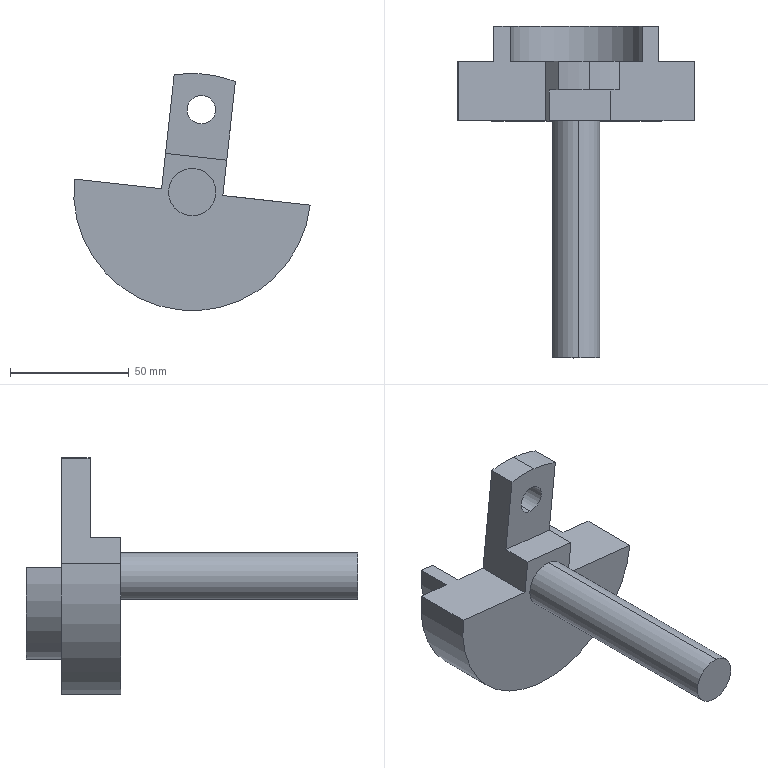Component | SolidWorks | Roller-5 | 1 solid | 20 faces | box 99.7 x 140 x 100 mm | volume 159117 mm3 | plane 11 | cylinder 9 | commonest cylinder face diameters 100 x3 12 x2 20 x2 56 x1 70 x1
build123d program:
from build123d import *

# Parameters (mm, degrees)
SKETCH2_W      = 83.89
SKETCH2_H      = 46.873
EXTRUDE2_DEPTH = 15
SKETCH3_W      = 56.676
SKETCH3_H      = 55.605
EXTRUDE3_DEPTH = 144.614
SKETCH4_R      = 6
EXTRUDE4_DEPTH = 144.614
SKETCH5_W      = 35
SKETCH5_H      = 13
EXTRUDE5_DEPTH = 117.402


with BuildPart() as part:
    # Sketch1 → Revolve1 (revolve)
    with BuildSketch(Plane.XY, mode=Mode.PRIVATE) as revolve1_sk:
        Polygon((0, 69.146), (28, 69.146), (28, 84.146), (35, 84.146), (35, 69.146), (50, 69.146), (50, 44.146), (10, 44.146), (10, -55.854), (0, -55.854), align=None)
    revolve(revolve1_sk.sketch.rotate(Axis((0, 0, 0), (0, 1, 0)), 90), axis=Axis((0, 0, 0), (0, 1, 0)))

    # Sketch2 → Extrude2 (cut)
    with BuildSketch(Plane(origin=(0, 84.146, 0), x_dir=(1, 0, 0), z_dir=(0, 1, 0))):
        with Locations((-6.945, 23.437)):
            Rectangle(SKETCH2_W, SKETCH2_H)
    extrude(amount=-EXTRUDE2_DEPTH, mode=Mode.SUBTRACT)

    # Sketch3 → Extrude3 (cut, through all)
    with BuildSketch(Plane(origin=(0, 69.146, 0), x_dir=(1, 0, 0), z_dir=(0, 1, 0))):
        with Locations((-41.338, 27.803)):
            Rectangle(SKETCH3_W, SKETCH3_H)
        with Locations((41.338, 27.803)):
            Rectangle(SKETCH3_W, SKETCH3_H)
    extrude(amount=-EXTRUDE3_DEPTH, mode=Mode.SUBTRACT)

    # Sketch4 → Extrude4 (cut, through all)
    with BuildSketch(Plane(origin=(0, 69.146, 0), x_dir=(1, 0, 0), z_dir=(0, 1, 0))):
        with Locations(Location((0, 35, 0), (0, 0, 270))):
            Circle(SKETCH4_R)
    extrude(amount=-EXTRUDE4_DEPTH, mode=Mode.SUBTRACT)

    # Sketch5 → Extrude5 (cut, through all)
    with BuildSketch(Plane(origin=(13, 0, 0), x_dir=(0, 0, -1), z_dir=(1, 0, 0))):
        with Locations((32.5, 50.646)):
            Rectangle(SKETCH5_W, SKETCH5_H)
    extrude(amount=-EXTRUDE5_DEPTH, mode=Mode.SUBTRACT)


solid = part.part

# Placed as in the assembly
solid = solid.moved(Location((-214.784, 444.838, 163), (180, -6.299, 180)))
STEP:
#1=COLOUR_RGB('',0.7922,0.8196,0.9333);
#2=FILL_AREA_STYLE_COLOUR('',#1);
#3=FILL_AREA_STYLE('',(#2));
#4=SURFACE_STYLE_FILL_AREA(#3);
#5=SURFACE_SIDE_STYLE('',(#4));
#6=SURFACE_STYLE_USAGE(.BOTH.,#5);
#7=PRESENTATION_STYLE_ASSIGNMENT((#6));
#8=CARTESIAN_POINT('',(-8.331,19.763,7.552));
#9=VERTEX_POINT('',#8);
#10=CARTESIAN_POINT('',(-8.279,19.763,8.022));
#11=VERTEX_POINT('',#10);
#12=CARTESIAN_POINT('',(-8.305,19.763,7.787));
#13=DIRECTION('',(0.,-1.,0.));
#14=DIRECTION('',(-0.1097,0.,-0.994));
#15=AXIS2_PLACEMENT_3D('',#12,#13,#14);
#16=CIRCLE('',#15,0.2362);
#17=EDGE_CURVE('',#9,#11,#16,.T.);
#18=ORIENTED_EDGE('',*,*,#17,.T.);
#19=CARTESIAN_POINT('',(-8.279,20.236,8.022));
#20=VERTEX_POINT('',#19);
#21=CARTESIAN_POINT('',(-8.279,15.314,8.022));
#22=DIRECTION('',(-0.,1.,-0.));
#23=VECTOR('',#22,39.37);
#24=LINE('',#21,#23);
#25=EDGE_CURVE('',#11,#20,#24,.T.);
#26=ORIENTED_EDGE('',*,*,#25,.T.);
#27=CARTESIAN_POINT('',(-8.331,20.236,7.552));
#28=VERTEX_POINT('',#27);
#29=CARTESIAN_POINT('',(-8.305,20.236,7.787));
#30=DIRECTION('',(-0.,1.,-0.));
#31=DIRECTION('',(-0.1097,0.,-0.994));
#32=AXIS2_PLACEMENT_3D('',#29,#30,#31);
#33=CIRCLE('',#32,0.2362);
#34=EDGE_CURVE('',#20,#28,#33,.T.);
#35=ORIENTED_EDGE('',*,*,#34,.T.);
#36=CARTESIAN_POINT('',(-8.331,15.314,7.552));
#37=DIRECTION('',(-0.,1.,-0.));
#38=VECTOR('',#37,39.37);
#39=LINE('',#36,#38);
#40=EDGE_CURVE('',#9,#28,#39,.T.);
#41=ORIENTED_EDGE('',*,*,#40,.F.);
#42=EDGE_LOOP('',(#18,#26,#35,#41));
#43=FACE_OUTER_BOUND('',#42,.T.);
#44=CARTESIAN_POINT('',(-8.305,15.314,7.787));
#45=DIRECTION('',(-0.,1.,-0.));
#46=DIRECTION('',(-0.1097,0.,-0.994));
#47=AXIS2_PLACEMENT_3D('',#44,#45,#46);
#48=CYLINDRICAL_SURFACE('',#47,0.2362);
#49=ADVANCED_FACE('',(#43),#48,.F.);
#50=CARTESIAN_POINT('',(-8.413,19.251,6.809));
#51=VERTEX_POINT('',#50);
#52=CARTESIAN_POINT('',(-8.499,19.251,6.026));
#53=VERTEX_POINT('',#52);
#54=CARTESIAN_POINT('',(-8.456,19.251,6.417));
#55=DIRECTION('',(0.,-1.,0.));
#56=DIRECTION('',(0.1097,0.,0.994));
#57=AXIS2_PLACEMENT_3D('',#54,#55,#56);
#58=CIRCLE('',#57,0.3937);
#59=EDGE_CURVE('',#51,#53,#58,.T.);
#60=ORIENTED_EDGE('',*,*,#59,.T.);
#61=CARTESIAN_POINT('',(-8.499,15.314,6.026));
#62=VERTEX_POINT('',#61);
#63=CARTESIAN_POINT('',(-8.499,17.513,6.026));
#64=DIRECTION('',(0.,-1.,0.));
#65=VECTOR('',#64,39.37);
#66=LINE('',#63,#65);
#67=EDGE_CURVE('',#53,#62,#66,.T.);
#68=ORIENTED_EDGE('',*,*,#67,.T.);
#69=CARTESIAN_POINT('',(-8.413,15.314,6.809));
#70=VERTEX_POINT('',#69);
#71=CARTESIAN_POINT('',(-8.456,15.314,6.417));
#72=DIRECTION('',(0.,-1.,0.));
#73=DIRECTION('',(0.1097,0.,0.994));
#74=AXIS2_PLACEMENT_3D('',#71,#72,#73);
#75=CIRCLE('',#74,0.3937);
#76=EDGE_CURVE('',#70,#62,#75,.T.);
#77=ORIENTED_EDGE('',*,*,#76,.F.);
#78=CARTESIAN_POINT('',(-8.413,17.513,6.809));
#79=DIRECTION('',(0.,-1.,0.));
#80=VECTOR('',#79,39.37);
#81=LINE('',#78,#80);
#82=EDGE_CURVE('',#51,#70,#81,.T.);
#83=ORIENTED_EDGE('',*,*,#82,.F.);
#84=EDGE_LOOP('',(#60,#68,#77,#83));
#85=FACE_OUTER_BOUND('',#84,.T.);
#86=CARTESIAN_POINT('',(-8.456,17.513,6.417));
#87=DIRECTION('',(0.,-1.,0.));
#88=DIRECTION('',(0.1097,0.,0.994));
#89=AXIS2_PLACEMENT_3D('',#86,#87,#88);
#90=CYLINDRICAL_SURFACE('',#89,0.3937);
#91=ADVANCED_FACE('',(#85),#90,.T.);
#92=CARTESIAN_POINT('',(-7.739,20.236,8.25));
#93=VERTEX_POINT('',#92);
#94=CARTESIAN_POINT('',(-8.24,20.236,8.374));
#95=VERTEX_POINT('',#94);
#96=CARTESIAN_POINT('',(-8.456,20.236,6.417));
#97=DIRECTION('',(0.,-1.,0.));
#98=DIRECTION('',(0.1097,0.,0.994));
#99=AXIS2_PLACEMENT_3D('',#96,#97,#98);
#100=CIRCLE('',#99,1.969);
#101=EDGE_CURVE('',#93,#95,#100,.T.);
#102=ORIENTED_EDGE('',*,*,#101,.T.);
#103=CARTESIAN_POINT('',(-8.24,19.763,8.374));
#104=VERTEX_POINT('',#103);
#105=CARTESIAN_POINT('',(-8.24,17.513,8.374));
#106=DIRECTION('',(0.,-1.,0.));
#107=VECTOR('',#106,39.37);
#108=LINE('',#105,#107);
#109=EDGE_CURVE('',#95,#104,#108,.T.);
#110=ORIENTED_EDGE('',*,*,#109,.T.);
#111=CARTESIAN_POINT('',(-7.739,19.763,8.25));
#112=VERTEX_POINT('',#111);
#113=CARTESIAN_POINT('',(-8.456,19.763,6.417));
#114=DIRECTION('',(0.,-1.,0.));
#115=DIRECTION('',(-0.1097,0.,-0.994));
#116=AXIS2_PLACEMENT_3D('',#113,#114,#115);
#117=CIRCLE('',#116,1.969);
#118=EDGE_CURVE('',#112,#104,#117,.T.);
#119=ORIENTED_EDGE('',*,*,#118,.F.);
#120=CARTESIAN_POINT('',(-7.739,17.513,8.25));
#121=DIRECTION('',(0.,-1.,0.));
#122=VECTOR('',#121,39.37);
#123=LINE('',#120,#122);
#124=EDGE_CURVE('',#93,#112,#123,.T.);
#125=ORIENTED_EDGE('',*,*,#124,.F.);
#126=EDGE_LOOP('',(#102,#110,#119,#125));
#127=FACE_OUTER_BOUND('',#126,.T.);
#128=CARTESIAN_POINT('',(-8.456,17.513,6.417));
#129=DIRECTION('',(0.,-1.,0.));
#130=DIRECTION('',(0.1097,0.,0.994));
#131=AXIS2_PLACEMENT_3D('',#128,#129,#130);
#132=CYLINDRICAL_SURFACE('',#131,1.969);
#133=ADVANCED_FACE('',(#127),#132,.T.);
#134=CARTESIAN_POINT('',(-9.826,20.236,6.569));
#135=VERTEX_POINT('',#134);
#136=CARTESIAN_POINT('',(-10.413,20.236,6.633));
#137=VERTEX_POINT('',#136);
#138=CARTESIAN_POINT('',(-11.183,20.236,6.718));
#139=DIRECTION('',(-0.994,-0.,0.1097));
#140=VECTOR('',#139,39.37);
#141=LINE('',#138,#140);
#142=EDGE_CURVE('',#135,#137,#141,.T.);
#143=ORIENTED_EDGE('',*,*,#142,.F.);
#144=CARTESIAN_POINT('',(-7.086,20.236,6.266));
#145=VERTEX_POINT('',#144);
#146=CARTESIAN_POINT('',(-8.456,20.236,6.417));
#147=DIRECTION('',(0.,-1.,0.));
#148=DIRECTION('',(0.1097,0.,0.994));
#149=AXIS2_PLACEMENT_3D('',#146,#147,#148);
#150=CIRCLE('',#149,1.378);
#151=EDGE_CURVE('',#135,#145,#150,.T.);
#152=ORIENTED_EDGE('',*,*,#151,.T.);
#153=CARTESIAN_POINT('',(-6.499,20.236,6.201));
#154=VERTEX_POINT('',#153);
#155=CARTESIAN_POINT('',(-5.729,20.236,6.116));
#156=DIRECTION('',(-0.994,-0.,0.1097));
#157=VECTOR('',#156,39.37);
#158=LINE('',#155,#157);
#159=EDGE_CURVE('',#154,#145,#158,.T.);
#160=ORIENTED_EDGE('',*,*,#159,.F.);
#161=CARTESIAN_POINT('',(-8.456,20.236,6.417));
#162=DIRECTION('',(0.,-1.,0.));
#163=DIRECTION('',(0.1097,0.,0.994));
#164=AXIS2_PLACEMENT_3D('',#161,#162,#163);
#165=CIRCLE('',#164,1.969);
#166=EDGE_CURVE('',#137,#154,#165,.T.);
#167=ORIENTED_EDGE('',*,*,#166,.F.);
#168=EDGE_LOOP('',(#143,#152,#160,#167));
#169=FACE_OUTER_BOUND('',#168,.T.);
#170=CARTESIAN_POINT('',(-9.826,20.236,6.569));
#171=DIRECTION('',(-0.,1.,-0.));
#172=DIRECTION('',(-0.1097,-0.,-0.994));
#173=AXIS2_PLACEMENT_3D('',#170,#171,#172);
#174=PLANE('',#173);
#175=ADVANCED_FACE('',(#169),#174,.T.);
#176=CARTESIAN_POINT('',(-10.413,19.251,6.633));
#177=VERTEX_POINT('',#176);
#178=CARTESIAN_POINT('',(-10.413,17.513,6.633));
#179=DIRECTION('',(0.,-1.,0.));
#180=VECTOR('',#179,39.37);
#181=LINE('',#178,#180);
#182=EDGE_CURVE('',#137,#177,#181,.T.);
#183=ORIENTED_EDGE('',*,*,#182,.F.);
#184=ORIENTED_EDGE('',*,*,#166,.T.);
#185=CARTESIAN_POINT('',(-6.499,19.251,6.201));
#186=VERTEX_POINT('',#185);
#187=CARTESIAN_POINT('',(-6.499,17.513,6.201));
#188=DIRECTION('',(-0.,1.,-0.));
#189=VECTOR('',#188,39.37);
#190=LINE('',#187,#189);
#191=EDGE_CURVE('',#186,#154,#190,.T.);
#192=ORIENTED_EDGE('',*,*,#191,.F.);
#193=CARTESIAN_POINT('',(-8.456,19.251,6.417));
#194=DIRECTION('',(0.,-1.,0.));
#195=DIRECTION('',(0.1097,0.,0.994));
#196=AXIS2_PLACEMENT_3D('',#193,#194,#195);
#197=CIRCLE('',#196,1.969);
#198=EDGE_CURVE('',#177,#186,#197,.T.);
#199=ORIENTED_EDGE('',*,*,#198,.F.);
#200=EDGE_LOOP('',(#183,#184,#192,#199));
#201=FACE_OUTER_BOUND('',#200,.T.);
#202=CARTESIAN_POINT('',(-8.456,17.513,6.417));
#203=DIRECTION('',(0.,-1.,0.));
#204=DIRECTION('',(0.1097,0.,0.994));
#205=AXIS2_PLACEMENT_3D('',#202,#203,#204);
#206=CYLINDRICAL_SURFACE('',#205,1.969);
#207=ADVANCED_FACE('',(#201),#206,.T.);
#208=CARTESIAN_POINT('',(-7.36,20.826,6.296));
#209=VERTEX_POINT('',#208);
#210=CARTESIAN_POINT('',(-7.36,20.236,6.296));
#211=VERTEX_POINT('',#210);
#212=CARTESIAN_POINT('',(-7.36,17.513,6.296));
#213=DIRECTION('',(0.,-1.,0.));
#214=VECTOR('',#213,39.37);
#215=LINE('',#212,#214);
#216=EDGE_CURVE('',#209,#211,#215,.T.);
#217=ORIENTED_EDGE('',*,*,#216,.F.);
#218=CARTESIAN_POINT('',(-9.552,20.826,6.538));
#219=VERTEX_POINT('',#218);
#220=CARTESIAN_POINT('',(-8.456,20.826,6.417));
#221=DIRECTION('',(0.,-1.,0.));
#222=DIRECTION('',(0.1097,0.,0.994));
#223=AXIS2_PLACEMENT_3D('',#220,#221,#222);
#224=CIRCLE('',#223,1.102);
#225=EDGE_CURVE('',#219,#209,#224,.T.);
#226=ORIENTED_EDGE('',*,*,#225,.F.);
#227=CARTESIAN_POINT('',(-9.552,20.236,6.538));
#228=VERTEX_POINT('',#227);
#229=CARTESIAN_POINT('',(-9.552,17.513,6.538));
#230=DIRECTION('',(-0.,1.,-0.));
#231=VECTOR('',#230,39.37);
#232=LINE('',#229,#231);
#233=EDGE_CURVE('',#228,#219,#232,.T.);
#234=ORIENTED_EDGE('',*,*,#233,.F.);
#235=CARTESIAN_POINT('',(-8.456,20.236,6.417));
#236=DIRECTION('',(0.,-1.,0.));
#237=DIRECTION('',(0.1097,0.,0.994));
#238=AXIS2_PLACEMENT_3D('',#235,#236,#237);
#239=CIRCLE('',#238,1.102);
#240=EDGE_CURVE('',#228,#211,#239,.T.);
#241=ORIENTED_EDGE('',*,*,#240,.T.);
#242=EDGE_LOOP('',(#217,#226,#234,#241));
#243=FACE_OUTER_BOUND('',#242,.T.);
#244=CARTESIAN_POINT('',(-8.456,17.513,6.417));
#245=DIRECTION('',(0.,-1.,0.));
#246=DIRECTION('',(0.1097,0.,0.994));
#247=AXIS2_PLACEMENT_3D('',#244,#245,#246);
#248=CYLINDRICAL_SURFACE('',#247,1.102);
#249=ADVANCED_FACE('',(#243),#248,.F.);
#250=CARTESIAN_POINT('',(-7.086,20.826,6.266));
#251=VERTEX_POINT('',#250);
#252=CARTESIAN_POINT('',(-6.543,20.826,6.206));
#253=DIRECTION('',(-0.994,-0.,0.1097));
#254=VECTOR('',#253,39.37);
#255=LINE('',#252,#254);
#256=EDGE_CURVE('',#251,#209,#255,.T.);
#257=ORIENTED_EDGE('',*,*,#256,.F.);
#258=CARTESIAN_POINT('',(-9.826,20.826,6.569));
#259=VERTEX_POINT('',#258);
#260=CARTESIAN_POINT('',(-8.456,20.826,6.417));
#261=DIRECTION('',(0.,-1.,0.));
#262=DIRECTION('',(0.1097,0.,0.994));
#263=AXIS2_PLACEMENT_3D('',#260,#261,#262);
#264=CIRCLE('',#263,1.378);
#265=EDGE_CURVE('',#259,#251,#264,.T.);
#266=ORIENTED_EDGE('',*,*,#265,.F.);
#267=CARTESIAN_POINT('',(-6.543,20.826,6.206));
#268=DIRECTION('',(-0.994,-0.,0.1097));
#269=VECTOR('',#268,39.37);
#270=LINE('',#267,#269);
#271=EDGE_CURVE('',#219,#259,#270,.T.);
#272=ORIENTED_EDGE('',*,*,#271,.F.);
#273=ORIENTED_EDGE('',*,*,#225,.T.);
#274=EDGE_LOOP('',(#257,#266,#272,#273));
#275=FACE_OUTER_BOUND('',#274,.T.);
#276=CARTESIAN_POINT('',(-9.552,20.826,6.538));
#277=DIRECTION('',(-0.,1.,-0.));
#278=DIRECTION('',(-0.1097,-0.,-0.994));
#279=AXIS2_PLACEMENT_3D('',#276,#277,#278);
#280=PLANE('',#279);
#281=ADVANCED_FACE('',(#275),#280,.T.);
#282=CARTESIAN_POINT('',(-7.086,17.513,6.266));
#283=DIRECTION('',(-0.,1.,-0.));
#284=VECTOR('',#283,39.37);
#285=LINE('',#282,#284);
#286=EDGE_CURVE('',#145,#251,#285,.T.);
#287=ORIENTED_EDGE('',*,*,#286,.F.);
#288=ORIENTED_EDGE('',*,*,#151,.F.);
#289=CARTESIAN_POINT('',(-9.826,16.452,6.569));
#290=DIRECTION('',(-0.,1.,-0.));
#291=VECTOR('',#290,39.37);
#292=LINE('',#289,#291);
#293=EDGE_CURVE('',#135,#259,#292,.T.);
#294=ORIENTED_EDGE('',*,*,#293,.T.);
#295=ORIENTED_EDGE('',*,*,#265,.T.);
#296=EDGE_LOOP('',(#287,#288,#294,#295));
#297=FACE_OUTER_BOUND('',#296,.T.);
#298=CARTESIAN_POINT('',(-8.456,17.513,6.417));
#299=DIRECTION('',(0.,-1.,0.));
#300=DIRECTION('',(0.1097,0.,0.994));
#301=AXIS2_PLACEMENT_3D('',#298,#299,#300);
#302=CYLINDRICAL_SURFACE('',#301,1.378);
#303=ADVANCED_FACE('',(#297),#302,.T.);
#304=CARTESIAN_POINT('',(-8.305,20.236,7.787));
#305=DIRECTION('',(-0.,1.,-0.));
#306=DIRECTION('',(-0.1097,0.,-0.994));
#307=AXIS2_PLACEMENT_3D('',#304,#305,#306);
#308=CIRCLE('',#307,0.2362);
#309=EDGE_CURVE('',#28,#20,#308,.T.);
#310=ORIENTED_EDGE('',*,*,#309,.F.);
#311=ORIENTED_EDGE('',*,*,#34,.F.);
#312=EDGE_LOOP('',(#310,#311));
#313=FACE_BOUND('',#312,.T.);
#314=CARTESIAN_POINT('',(-8.965,20.236,6.473));
#315=VERTEX_POINT('',#314);
#316=CARTESIAN_POINT('',(-11.183,20.236,6.718));
#317=DIRECTION('',(-0.994,-0.,0.1097));
#318=VECTOR('',#317,39.37);
#319=LINE('',#316,#318);
#320=EDGE_CURVE('',#315,#228,#319,.T.);
#321=ORIENTED_EDGE('',*,*,#320,.F.);
#322=CARTESIAN_POINT('',(-8.756,20.236,8.363));
#323=VERTEX_POINT('',#322);
#324=CARTESIAN_POINT('',(-8.725,20.236,8.649));
#325=DIRECTION('',(-0.1097,-0.,-0.994));
#326=VECTOR('',#325,39.37);
#327=LINE('',#324,#326);
#328=EDGE_CURVE('',#323,#315,#327,.T.);
#329=ORIENTED_EDGE('',*,*,#328,.F.);
#330=CARTESIAN_POINT('',(-8.456,20.236,6.417));
#331=DIRECTION('',(0.,-1.,0.));
#332=DIRECTION('',(0.1097,0.,0.994));
#333=AXIS2_PLACEMENT_3D('',#330,#331,#332);
#334=CIRCLE('',#333,1.969);
#335=EDGE_CURVE('',#95,#323,#334,.T.);
#336=ORIENTED_EDGE('',*,*,#335,.F.);
#337=ORIENTED_EDGE('',*,*,#101,.F.);
#338=CARTESIAN_POINT('',(-7.947,20.236,6.361));
#339=VERTEX_POINT('',#338);
#340=CARTESIAN_POINT('',(-7.707,20.236,8.537));
#341=DIRECTION('',(0.1097,0.,0.994));
#342=VECTOR('',#341,39.37);
#343=LINE('',#340,#342);
#344=EDGE_CURVE('',#339,#93,#343,.T.);
#345=ORIENTED_EDGE('',*,*,#344,.F.);
#346=CARTESIAN_POINT('',(-5.729,20.236,6.116));
#347=DIRECTION('',(-0.994,-0.,0.1097));
#348=VECTOR('',#347,39.37);
#349=LINE('',#346,#348);
#350=EDGE_CURVE('',#211,#339,#349,.T.);
#351=ORIENTED_EDGE('',*,*,#350,.F.);
#352=ORIENTED_EDGE('',*,*,#240,.F.);
#353=EDGE_LOOP('',(#321,#329,#336,#337,#345,#351,#352));
#354=FACE_OUTER_BOUND('',#353,.T.);
#355=CARTESIAN_POINT('',(-9.826,20.236,6.569));
#356=DIRECTION('',(-0.,1.,-0.));
#357=DIRECTION('',(-0.1097,-0.,-0.994));
#358=AXIS2_PLACEMENT_3D('',#355,#356,#357);
#359=PLANE('',#358);
#360=ADVANCED_FACE('',(#313,#354),#359,.T.);
#361=ORIENTED_EDGE('',*,*,#109,.F.);
#362=ORIENTED_EDGE('',*,*,#335,.T.);
#363=CARTESIAN_POINT('',(-8.756,19.763,8.363));
#364=VERTEX_POINT('',#363);
#365=CARTESIAN_POINT('',(-8.756,17.513,8.363));
#366=DIRECTION('',(-0.,1.,-0.));
#367=VECTOR('',#366,39.37);
#368=LINE('',#365,#367);
#369=EDGE_CURVE('',#364,#323,#368,.T.);
#370=ORIENTED_EDGE('',*,*,#369,.F.);
#371=CARTESIAN_POINT('',(-8.456,19.763,6.417));
#372=DIRECTION('',(0.,-1.,0.));
#373=DIRECTION('',(-0.1097,0.,-0.994));
#374=AXIS2_PLACEMENT_3D('',#371,#372,#373);
#375=CIRCLE('',#374,1.969);
#376=EDGE_CURVE('',#104,#364,#375,.T.);
#377=ORIENTED_EDGE('',*,*,#376,.F.);
#378=EDGE_LOOP('',(#361,#362,#370,#377));
#379=FACE_OUTER_BOUND('',#378,.T.);
#380=CARTESIAN_POINT('',(-8.456,17.513,6.417));
#381=DIRECTION('',(0.,-1.,0.));
#382=DIRECTION('',(0.1097,0.,0.994));
#383=AXIS2_PLACEMENT_3D('',#380,#381,#382);
#384=CYLINDRICAL_SURFACE('',#383,1.969);
#385=ADVANCED_FACE('',(#379),#384,.T.);
#386=CARTESIAN_POINT('',(-7.883,19.251,6.948));
#387=VERTEX_POINT('',#386);
#388=CARTESIAN_POINT('',(-8.9,19.251,7.06));
#389=VERTEX_POINT('',#388);
#390=CARTESIAN_POINT('',(-6.435,19.251,6.788));
#391=DIRECTION('',(-0.994,-0.,0.1097));
#392=VECTOR('',#391,39.37);
#393=LINE('',#390,#392);
#394=EDGE_CURVE('',#387,#389,#393,.T.);
#395=ORIENTED_EDGE('',*,*,#394,.T.);
#396=CARTESIAN_POINT('',(-8.965,19.251,6.473));
#397=VERTEX_POINT('',#396);
#398=CARTESIAN_POINT('',(-8.965,19.251,6.473));
#399=DIRECTION('',(0.1097,0.,0.994));
#400=VECTOR('',#399,39.37);
#401=LINE('',#398,#400);
#402=EDGE_CURVE('',#397,#389,#401,.T.);
#403=ORIENTED_EDGE('',*,*,#402,.F.);
#404=CARTESIAN_POINT('',(-10.413,19.251,6.633));
#405=DIRECTION('',(0.994,0.,-0.1097));
#406=VECTOR('',#405,39.37);
#407=LINE('',#404,#406);
#408=EDGE_CURVE('',#177,#397,#407,.T.);
#409=ORIENTED_EDGE('',*,*,#408,.F.);
#410=ORIENTED_EDGE('',*,*,#198,.T.);
#411=CARTESIAN_POINT('',(-7.947,19.251,6.361));
#412=VERTEX_POINT('',#411);
#413=CARTESIAN_POINT('',(-10.413,19.251,6.633));
#414=DIRECTION('',(0.994,0.,-0.1097));
#415=VECTOR('',#414,39.37);
#416=LINE('',#413,#415);
#417=EDGE_CURVE('',#412,#186,#416,.T.);
#418=ORIENTED_EDGE('',*,*,#417,.F.);
#419=CARTESIAN_POINT('',(-7.947,19.251,6.361));
#420=DIRECTION('',(-0.1097,-0.,-0.994));
#421=VECTOR('',#420,39.37);
#422=LINE('',#419,#421);
#423=EDGE_CURVE('',#387,#412,#422,.T.);
#424=ORIENTED_EDGE('',*,*,#423,.F.);
#425=EDGE_LOOP('',(#395,#403,#409,#410,#418,#424));
#426=FACE_OUTER_BOUND('',#425,.T.);
#427=ORIENTED_EDGE('',*,*,#59,.F.);
#428=CARTESIAN_POINT('',(-8.456,19.251,6.417));
#429=DIRECTION('',(0.,-1.,0.));
#430=DIRECTION('',(0.1097,0.,0.994));
#431=AXIS2_PLACEMENT_3D('',#428,#429,#430);
#432=CIRCLE('',#431,0.3937);
#433=EDGE_CURVE('',#53,#51,#432,.T.);
#434=ORIENTED_EDGE('',*,*,#433,.F.);
#435=EDGE_LOOP('',(#427,#434));
#436=FACE_BOUND('',#435,.T.);
#437=CARTESIAN_POINT('',(-10.413,19.251,6.633));
#438=DIRECTION('',(0.,-1.,0.));
#439=DIRECTION('',(0.1097,0.,0.994));
#440=AXIS2_PLACEMENT_3D('',#437,#438,#439);
#441=PLANE('',#440);
#442=ADVANCED_FACE('',(#426,#436),#441,.T.);
#443=ORIENTED_EDGE('',*,*,#67,.F.);
#444=ORIENTED_EDGE('',*,*,#433,.T.);
#445=ORIENTED_EDGE('',*,*,#82,.T.);
#446=CARTESIAN_POINT('',(-8.456,15.314,6.417));
#447=DIRECTION('',(0.,-1.,0.));
#448=DIRECTION('',(0.1097,0.,0.994));
#449=AXIS2_PLACEMENT_3D('',#446,#447,#448);
#450=CIRCLE('',#449,0.3937);
#451=EDGE_CURVE('',#62,#70,#450,.T.);
#452=ORIENTED_EDGE('',*,*,#451,.F.);
#453=EDGE_LOOP('',(#443,#444,#445,#452));
#454=FACE_OUTER_BOUND('',#453,.T.);
#455=CARTESIAN_POINT('',(-8.456,17.513,6.417));
#456=DIRECTION('',(0.,-1.,0.));
#457=DIRECTION('',(0.1097,0.,0.994));
#458=AXIS2_PLACEMENT_3D('',#455,#456,#457);
#459=CYLINDRICAL_SURFACE('',#458,0.3937);
#460=ADVANCED_FACE('',(#454),#459,.T.);
#461=ORIENTED_EDGE('',*,*,#76,.T.);
#462=ORIENTED_EDGE('',*,*,#451,.T.);
#463=EDGE_LOOP('',(#461,#462));
#464=FACE_OUTER_BOUND('',#463,.T.);
#465=CARTESIAN_POINT('',(-8.847,15.314,6.461));
#466=DIRECTION('',(0.,-1.,0.));
#467=DIRECTION('',(0.1097,0.,0.994));
#468=AXIS2_PLACEMENT_3D('',#465,#466,#467);
#469=PLANE('',#468);
#470=ADVANCED_FACE('',(#464),#469,.T.);
#471=ORIENTED_EDGE('',*,*,#216,.T.);
#472=ORIENTED_EDGE('',*,*,#350,.T.);
#473=CARTESIAN_POINT('',(-7.947,15.314,6.361));
#474=DIRECTION('',(-0.,1.,-0.));
#475=VECTOR('',#474,39.37);
#476=LINE('',#473,#475);
#477=EDGE_CURVE('',#412,#339,#476,.T.);
#478=ORIENTED_EDGE('',*,*,#477,.F.);
#479=ORIENTED_EDGE('',*,*,#417,.T.);
#480=ORIENTED_EDGE('',*,*,#191,.T.);
#481=ORIENTED_EDGE('',*,*,#159,.T.);
#482=ORIENTED_EDGE('',*,*,#286,.T.);
#483=ORIENTED_EDGE('',*,*,#256,.T.);
#484=EDGE_LOOP('',(#471,#472,#478,#479,#480,#481,#482,#483));
#485=FACE_OUTER_BOUND('',#484,.T.);
#486=CARTESIAN_POINT('',(-6.543,16.452,6.206));
#487=DIRECTION('',(-0.1097,-0.,-0.994));
#488=DIRECTION('',(-0.994,-0.,0.1097));
#489=AXIS2_PLACEMENT_3D('',#486,#487,#488);
#490=PLANE('',#489);
#491=ADVANCED_FACE('',(#485),#490,.F.);
#492=ORIENTED_EDGE('',*,*,#233,.T.);
#493=ORIENTED_EDGE('',*,*,#271,.T.);
#494=ORIENTED_EDGE('',*,*,#293,.F.);
#495=ORIENTED_EDGE('',*,*,#142,.T.);
#496=ORIENTED_EDGE('',*,*,#182,.T.);
#497=ORIENTED_EDGE('',*,*,#408,.T.);
#498=CARTESIAN_POINT('',(-8.965,15.314,6.473));
#499=DIRECTION('',(-0.,1.,-0.));
#500=VECTOR('',#499,39.37);
#501=LINE('',#498,#500);
#502=EDGE_CURVE('',#397,#315,#501,.T.);
#503=ORIENTED_EDGE('',*,*,#502,.T.);
#504=ORIENTED_EDGE('',*,*,#320,.T.);
#505=EDGE_LOOP('',(#492,#493,#494,#495,#496,#497,#503,#504));
#506=FACE_OUTER_BOUND('',#505,.T.);
#507=CARTESIAN_POINT('',(-6.543,16.452,6.206));
#508=DIRECTION('',(-0.1097,-0.,-0.994));
#509=DIRECTION('',(-0.994,-0.,0.1097));
#510=AXIS2_PLACEMENT_3D('',#507,#508,#509);
#511=PLANE('',#510);
#512=ADVANCED_FACE('',(#506),#511,.F.);
#513=CARTESIAN_POINT('',(-7.883,19.763,6.948));
#514=VERTEX_POINT('',#513);
#515=CARTESIAN_POINT('',(-7.707,19.763,8.537));
#516=DIRECTION('',(-0.1097,-0.,-0.994));
#517=VECTOR('',#516,39.37);
#518=LINE('',#515,#517);
#519=EDGE_CURVE('',#112,#514,#518,.T.);
#520=ORIENTED_EDGE('',*,*,#519,.T.);
#521=CARTESIAN_POINT('',(-7.883,15.314,6.948));
#522=DIRECTION('',(0.,-1.,0.));
#523=VECTOR('',#522,39.37);
#524=LINE('',#521,#523);
#525=EDGE_CURVE('',#514,#387,#524,.T.);
#526=ORIENTED_EDGE('',*,*,#525,.T.);
#527=ORIENTED_EDGE('',*,*,#423,.T.);
#528=ORIENTED_EDGE('',*,*,#477,.T.);
#529=ORIENTED_EDGE('',*,*,#344,.T.);
#530=ORIENTED_EDGE('',*,*,#124,.T.);
#531=EDGE_LOOP('',(#520,#526,#527,#528,#529,#530));
#532=FACE_OUTER_BOUND('',#531,.T.);
#533=CARTESIAN_POINT('',(-7.707,15.314,8.537));
#534=DIRECTION('',(-0.994,-0.,0.1097));
#535=DIRECTION('',(0.1097,0.,0.994));
#536=AXIS2_PLACEMENT_3D('',#533,#534,#535);
#537=PLANE('',#536);
#538=ADVANCED_FACE('',(#532),#537,.F.);
#539=ORIENTED_EDGE('',*,*,#402,.T.);
#540=CARTESIAN_POINT('',(-8.9,19.763,7.06));
#541=VERTEX_POINT('',#540);
#542=CARTESIAN_POINT('',(-8.9,19.251,7.06));
#543=DIRECTION('',(0.,-1.,0.));
#544=VECTOR('',#543,39.37);
#545=LINE('',#542,#544);
#546=EDGE_CURVE('',#541,#389,#545,.T.);
#547=ORIENTED_EDGE('',*,*,#546,.F.);
#548=CARTESIAN_POINT('',(-8.749,19.763,8.43));
#549=DIRECTION('',(-0.1097,-0.,-0.994));
#550=VECTOR('',#549,39.37);
#551=LINE('',#548,#550);
#552=EDGE_CURVE('',#364,#541,#551,.T.);
#553=ORIENTED_EDGE('',*,*,#552,.F.);
#554=ORIENTED_EDGE('',*,*,#369,.T.);
#555=ORIENTED_EDGE('',*,*,#328,.T.);
#556=ORIENTED_EDGE('',*,*,#502,.F.);
#557=EDGE_LOOP('',(#539,#547,#553,#554,#555,#556));
#558=FACE_OUTER_BOUND('',#557,.T.);
#559=CARTESIAN_POINT('',(-8.725,15.314,8.649));
#560=DIRECTION('',(0.994,0.,-0.1097));
#561=DIRECTION('',(-0.1097,-0.,-0.994));
#562=AXIS2_PLACEMENT_3D('',#559,#560,#561);
#563=PLANE('',#562);
#564=ADVANCED_FACE('',(#558),#563,.F.);
#565=ORIENTED_EDGE('',*,*,#25,.F.);
#566=CARTESIAN_POINT('',(-8.305,19.763,7.787));
#567=DIRECTION('',(0.,-1.,0.));
#568=DIRECTION('',(-0.1097,0.,-0.994));
#569=AXIS2_PLACEMENT_3D('',#566,#567,#568);
#570=CIRCLE('',#569,0.2362);
#571=EDGE_CURVE('',#11,#9,#570,.T.);
#572=ORIENTED_EDGE('',*,*,#571,.T.);
#573=ORIENTED_EDGE('',*,*,#40,.T.);
#574=ORIENTED_EDGE('',*,*,#309,.T.);
#575=EDGE_LOOP('',(#565,#572,#573,#574));
#576=FACE_OUTER_BOUND('',#575,.T.);
#577=CARTESIAN_POINT('',(-8.305,15.314,7.787));
#578=DIRECTION('',(-0.,1.,-0.));
#579=DIRECTION('',(-0.1097,0.,-0.994));
#580=AXIS2_PLACEMENT_3D('',#577,#578,#579);
#581=CYLINDRICAL_SURFACE('',#580,0.2362);
#582=ADVANCED_FACE('',(#576),#581,.F.);
#583=CARTESIAN_POINT('',(-6.435,19.763,6.788));
#584=DIRECTION('',(-0.994,-0.,0.1097));
#585=VECTOR('',#584,39.37);
#586=LINE('',#583,#585);
#587=EDGE_CURVE('',#514,#541,#586,.T.);
#588=ORIENTED_EDGE('',*,*,#587,.T.);
#589=ORIENTED_EDGE('',*,*,#546,.T.);
#590=ORIENTED_EDGE('',*,*,#394,.F.);
#591=ORIENTED_EDGE('',*,*,#525,.F.);
#592=EDGE_LOOP('',(#588,#589,#590,#591));
#593=FACE_OUTER_BOUND('',#592,.T.);
#594=CARTESIAN_POINT('',(-6.435,19.251,6.788));
#595=DIRECTION('',(-0.1097,-0.,-0.994));
#596=DIRECTION('',(-0.994,-0.,0.1097));
#597=AXIS2_PLACEMENT_3D('',#594,#595,#596);
#598=PLANE('',#597);
#599=ADVANCED_FACE('',(#593),#598,.F.);
#600=ORIENTED_EDGE('',*,*,#118,.T.);
#601=ORIENTED_EDGE('',*,*,#376,.T.);
#602=ORIENTED_EDGE('',*,*,#552,.T.);
#603=ORIENTED_EDGE('',*,*,#587,.F.);
#604=ORIENTED_EDGE('',*,*,#519,.F.);
#605=EDGE_LOOP('',(#600,#601,#602,#603,#604));
#606=FACE_OUTER_BOUND('',#605,.T.);
#607=ORIENTED_EDGE('',*,*,#17,.F.);
#608=ORIENTED_EDGE('',*,*,#571,.F.);
#609=EDGE_LOOP('',(#607,#608));
#610=FACE_BOUND('',#609,.T.);
#611=CARTESIAN_POINT('',(-6.283,19.763,8.158));
#612=DIRECTION('',(-0.,1.,-0.));
#613=DIRECTION('',(-0.1097,-0.,-0.994));
#614=AXIS2_PLACEMENT_3D('',#611,#612,#613);
#615=PLANE('',#614);
#616=ADVANCED_FACE('',(#606,#610),#615,.F.);
#617=CLOSED_SHELL('',(#49,#91,#133,#175,#207,#249,#281,#303,#360,#385,#442,#460,#470,#491,#512,#538,#564,#582,#599,#616));
#618=MANIFOLD_SOLID_BREP('',#617);
#619=STYLED_ITEM('',(#7),#618);
#620=PRESENTATION_LAYER_ASSIGNMENT('','',(#619));
#621=(LENGTH_UNIT()NAMED_UNIT(*)SI_UNIT($,.METRE.));
#622=LENGTH_MEASURE_WITH_UNIT(LENGTH_MEASURE(0.0254),#621);
#623=DIMENSIONAL_EXPONENTS(1.,0.,0.,0.,0.,0.,0.);
#624=(CONVERSION_BASED_UNIT('',#622)LENGTH_UNIT()NAMED_UNIT(#623));
#625=UNCERTAINTY_MEASURE_WITH_UNIT(LENGTH_MEASURE(0.00001),#624,'','');
#626=(NAMED_UNIT(*)PLANE_ANGLE_UNIT()SI_UNIT($,.RADIAN.));
#627=(NAMED_UNIT(*)SI_UNIT($,.STERADIAN.)SOLID_ANGLE_UNIT());
#628=(GEOMETRIC_REPRESENTATION_CONTEXT(3)GLOBAL_UNCERTAINTY_ASSIGNED_CONTEXT((#625))GLOBAL_UNIT_ASSIGNED_CONTEXT((#624,#626,#627))REPRESENTATION_CONTEXT('',''));
#629=MECHANICAL_DESIGN_GEOMETRIC_PRESENTATION_REPRESENTATION('',(#619),#628);
#630=CARTESIAN_POINT('',(0.,0.,0.));
#631=DIRECTION('',(0.,0.,1.));
#632=DIRECTION('',(1.,0.,0.));
#633=AXIS2_PLACEMENT_3D('',#630,#631,#632);
#634=(LENGTH_UNIT()NAMED_UNIT(*)SI_UNIT($,.METRE.));
#635=LENGTH_MEASURE_WITH_UNIT(LENGTH_MEASURE(0.0254),#634);
#636=DIMENSIONAL_EXPONENTS(1.,0.,0.,0.,0.,0.,0.);
#637=(CONVERSION_BASED_UNIT('',#635)LENGTH_UNIT()NAMED_UNIT(#636));
#638=UNCERTAINTY_MEASURE_WITH_UNIT(LENGTH_MEASURE(0.00001),#637,'','');
#639=(NAMED_UNIT(*)PLANE_ANGLE_UNIT()SI_UNIT($,.RADIAN.));
#640=(NAMED_UNIT(*)SI_UNIT($,.STERADIAN.)SOLID_ANGLE_UNIT());
#641=(GEOMETRIC_REPRESENTATION_CONTEXT(3)GLOBAL_UNCERTAINTY_ASSIGNED_CONTEXT((#638))GLOBAL_UNIT_ASSIGNED_CONTEXT((#637,#639,#640))REPRESENTATION_CONTEXT('',''));
#642=ADVANCED_BREP_SHAPE_REPRESENTATION('',(#618,#633),#641);